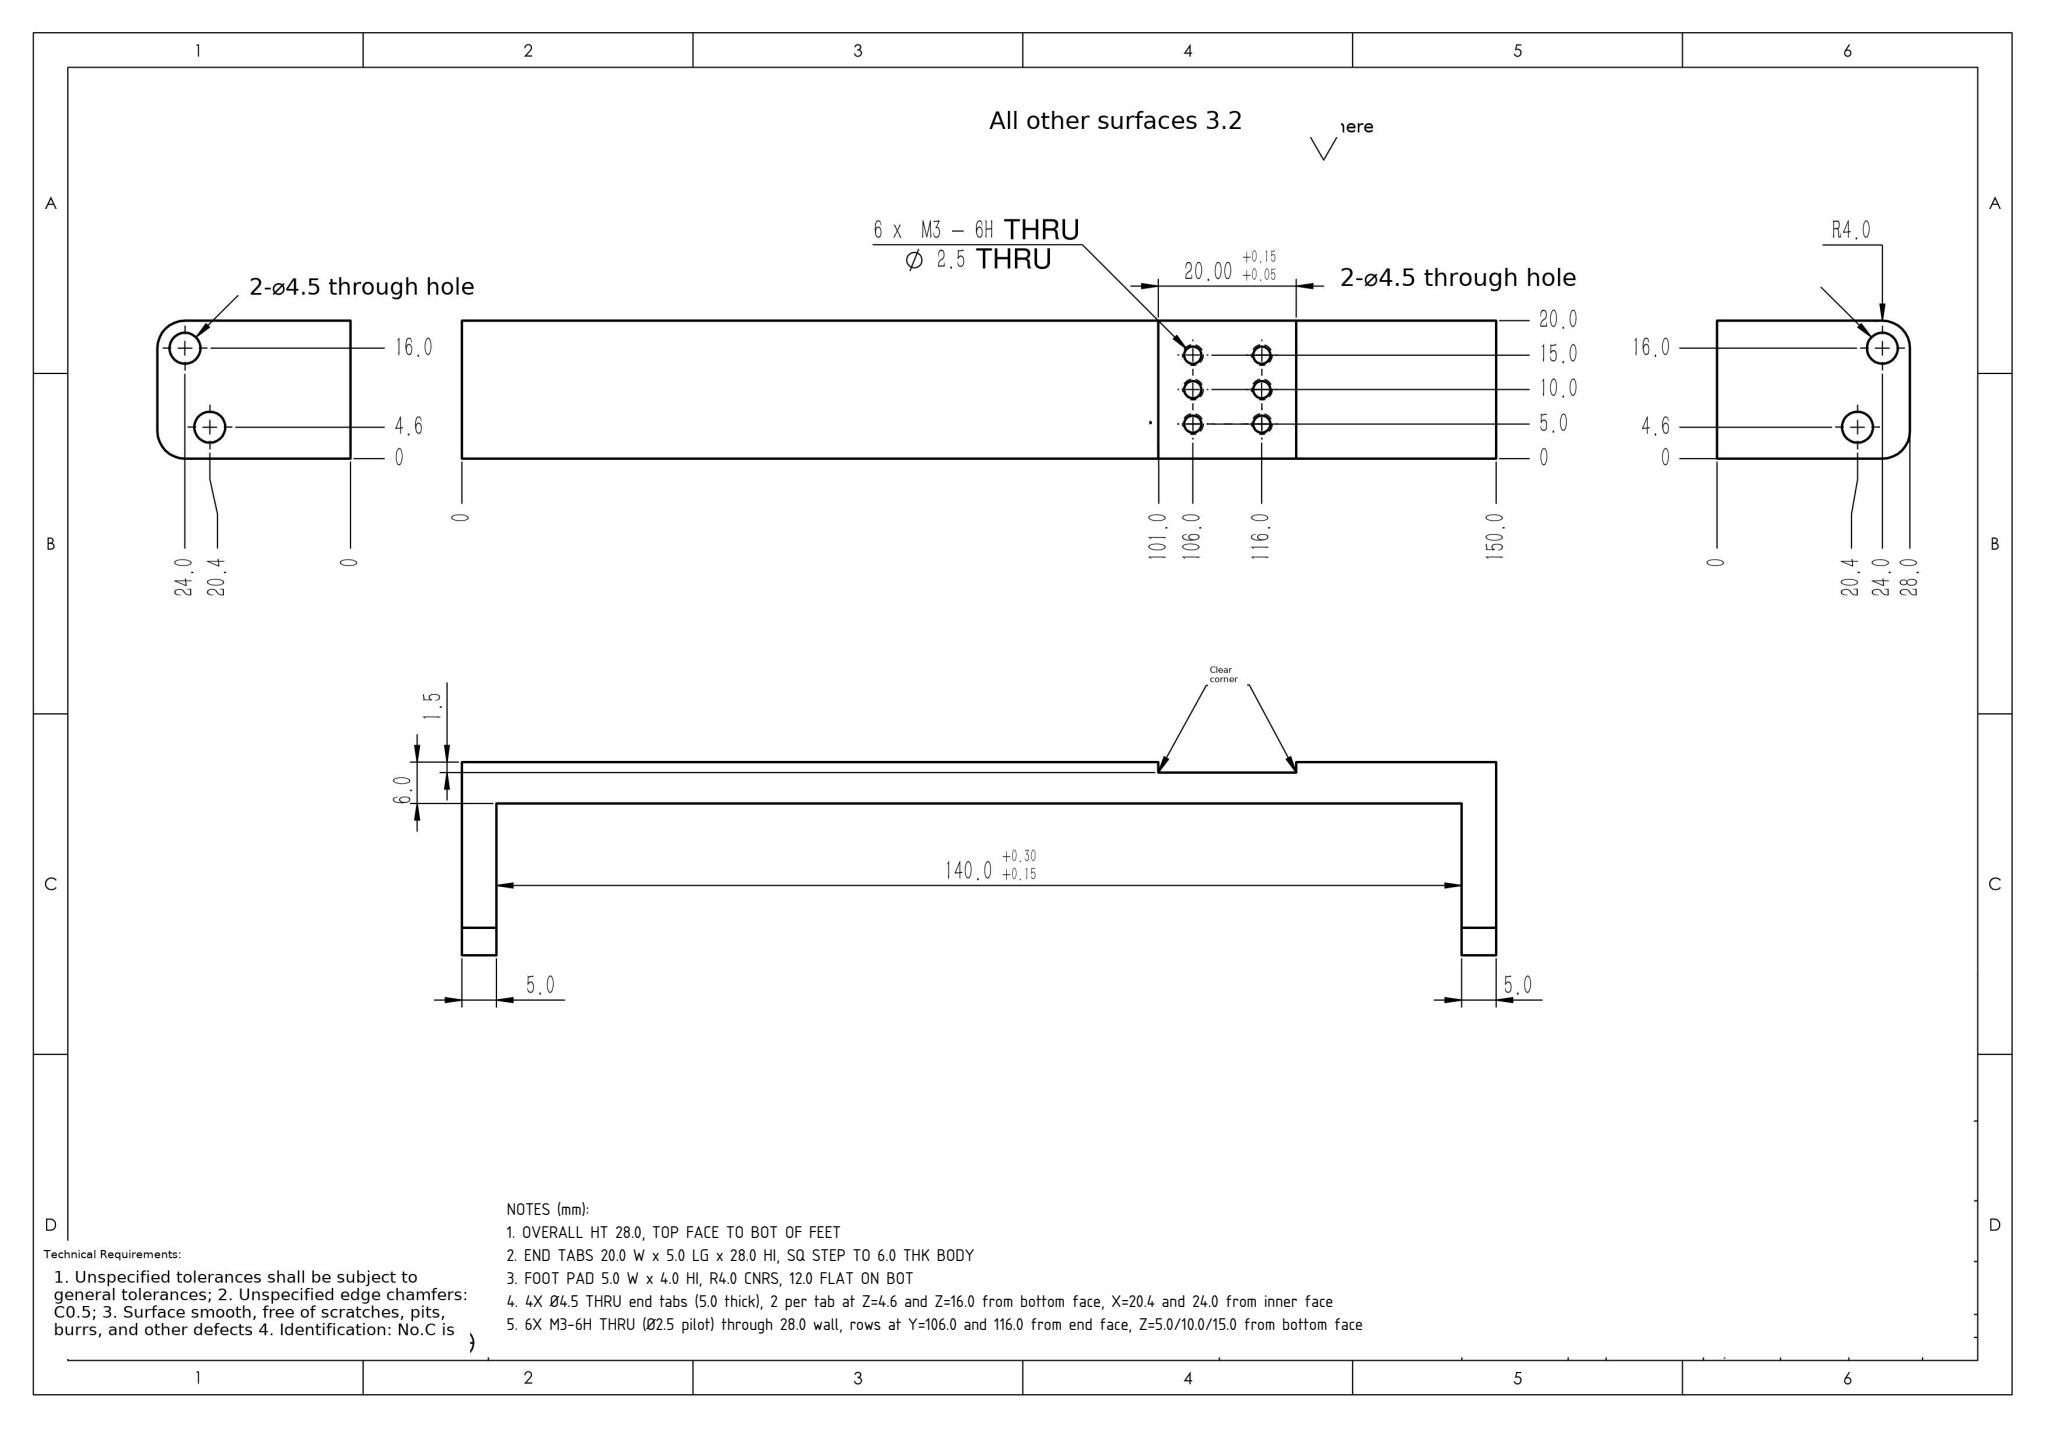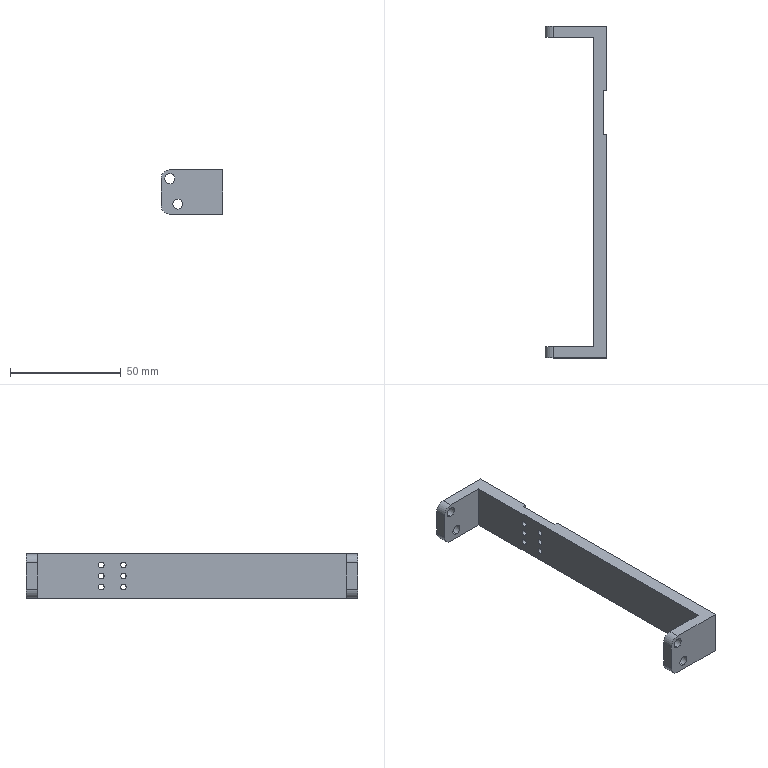Part | SolidWorks | mm | 1 solid | 46 faces | box 28 x 150 x 20 mm | volume 21281 mm3 | cylinder 24 | plane 22 | commonest cylinder face diameters 2.5 x12 4.5 x8 8 x4
Drawing notes:
OVERALL HT 28.0, TOP FACE TO BOT OF FEET | from the solid: bbox_xyz x = 28.0; x planes at 0.0 (foot bottoms) and 28.0 (top face)
END TABS 20.0 W x 5.0 LG x 28.0 HI, SQ STEP TO 6.0 THK BODY | from the solid: z 0-20 at tabs; y planes 0/5 and 145/150 = 5.0 lg; tabs x 0-28 vs body x 22.0-28.0 = 6.0 thk; no cones
FOOT PAD 5.0 W x 4.0 HI, R4.0 CNRS, 12.0 FLAT ON BOT | from the solid: legs y 0-5 & 145-150 = 5.0 W; Ø8.0 cyls axis y at x=4.0, z=4.0 & 16.0 -> flat z 4-16 = 12.0
4X Ø4.5 THRU end tabs (5.0 thick), 2 per tab at Z=4.6 and Z=16.0 from bottom face, X=20.4 and 24.0 from inner face | from the solid: cylinders [4.5,"y",[4.0,null,16.0],5.0] and [4.5,"y",[7.61,null,4.56],5.0]; y-planes 0.0/5.0 and 145.0/150.0
6X M3-6H THRU (Ø2.5 pilot) through 28.0 wall, rows at Y=106.0 and 116.0 from end face, Z=5.0/10.0/15.0 from bottom face | from the solid: cylinders 2.5 dia, axis x, at y=106.0/116.0 and z=5.0/10.0/15.0, length 4.5